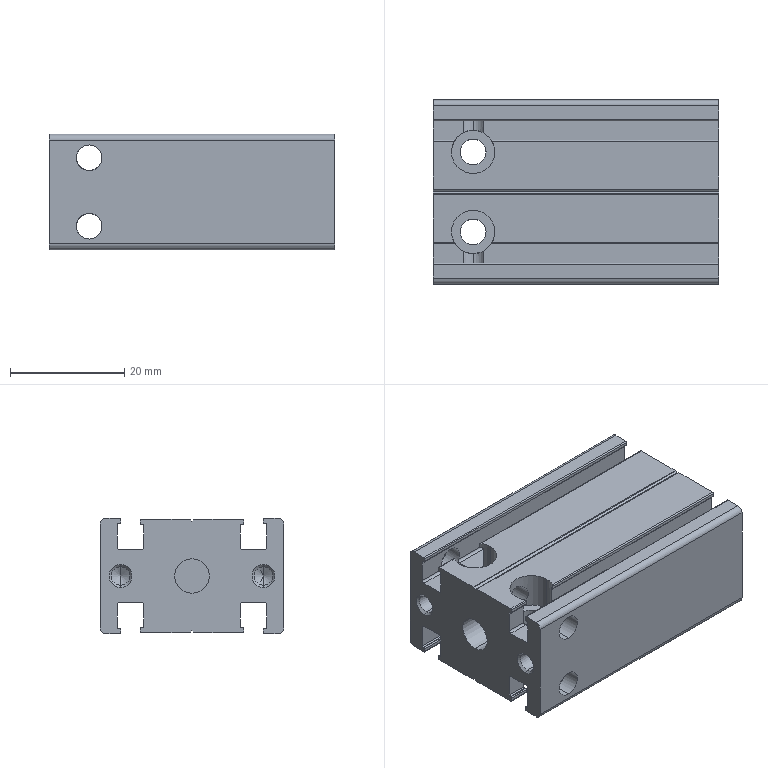Component | SolidWorks | 09MD-16x10-S (0)-1_09MD 16x10-S10 - Body-1 | 1 solid | 206 faces | volume 20614 mm3 | cylinder 114 | plane 72 | cone 20 | commonest cylinder face diameters 0.4 x40 4.5 x16 0.8 x16 7.6 x8 3.242 x8 3 x6 1.43 x4 4.134 x4